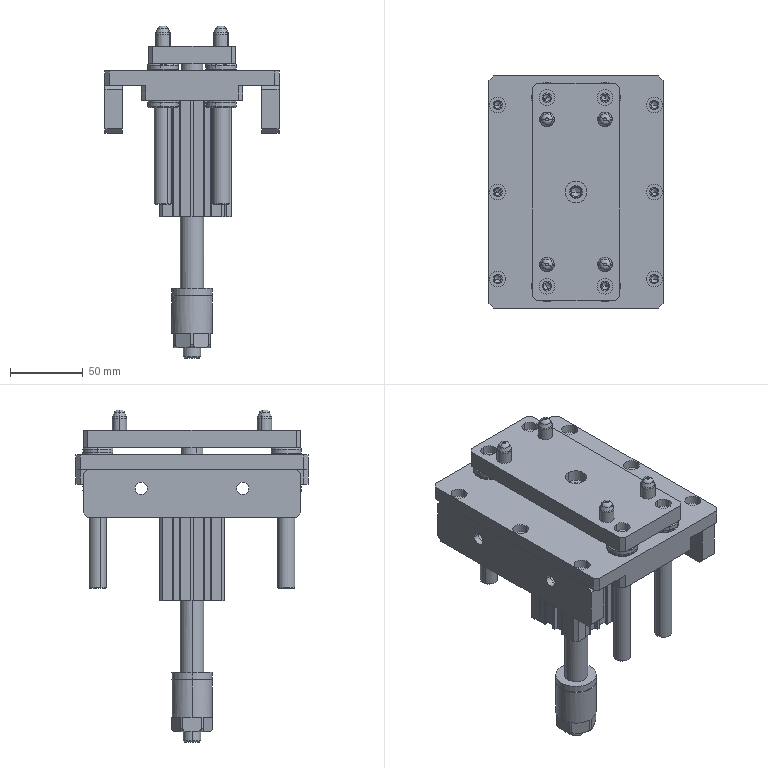Assembly | SolidWorks | mm | 20 component files | 20 solids | 847 faces | box 120 x 160 x 228.9 mm | volume 634230 mm3 | cylinder 377 | plane 268 | cone 138 | torus 48 | spline 16 | commonest cylinder face diameters 11 x36 0.4 x36 21 x32 12 x28 6.6 x24 5 x20 9 x18 10 x16
Bill of materials:
A-C13SupportCylinderBasePlate | 1 |  | Rectangular plate with chamfered corners. It has a stepped underside, a central counterbored through hole, four small holes around the center, four large counterbored holes near the ends and six small holes along the long edges.
A-C14LocatingMechanismGuidePost | 4 |  | Long slender round rod with a small axial hole at one end. It may be a hollow tube.
A-C15UpperSupportPlate | 1 |  | Long rectangular flat plate with chamfered corners. It has eight counterbored holes in two-by-two groups at each end and one central counterbored hole.
A-C17GuidePin | 4 |  | Solid cylinder with a rounded, tapered, dome-like end and a small chamfer at the opposite end.
A-C18EjectorMechanismConnectingBlock2 | 2 |  | Rectangular bar with chamfered end corners. Two larger holes pass through the wide face and three small holes are on one narrow face.
BEN | 1 |  | Square-section extruded-profile body. It has a large central bore, four corner bores, slots and grooves running along its length, a raised tab on one side, and two cross holes in one side face.
GAN | 1 |  | Stepped round shaft with a short collar section made of several flanges. It has an axial hole at one end and cross features near the ends.
TIAO | 1 |  | Cylindrical sleeve with an axial through bore and a thin circumferential line/groove near one end. The opposite end has a section with wrench-style flats.
LinearBearingLMUM12 | 4 |  | Thick-walled cylindrical bushing with an axial through bore, rounded edges, and two external circumferential grooves near the ends.
Mates:
1. coincident | A-C14LocatingMechanismGuidePost-1 face at (-53.181, -42.432, 18) dir (0, 0, 1) | A-C14LocatingMechanismGuidePost-2 face at (-53.181, 87.568, 18) dir (0, 0, 1)
2. concentric | A-C14LocatingMechanismGuidePost-1 face at (-53.181, -42.432, 18) dir (0, 0, 1) r 2.5 | A-C15UpperSupportPlate-1 face at (-53.181, -42.432, 27) dir (0, 0, 1) r 3.3
3. concentric | A-C13SupportCylinderBasePlate-1 face at (-53.181, 87.568, 10) dir (0, 0, -1) r 10.6 | LinearBearingLMUM12-1 face at (-53.181, 87.568, 14.9) dir (0, 0, -1) r 10.5
4. coincident | A-C13SupportCylinderBasePlate-1 face at (-68.181, 102.568, -10.3) dir (0, 0, -1) | LinearBearingLMUM12-1 face at (-53.181, 77.068, -10.3) dir (0, 0, -1)
5. concentric | A-C13SupportCylinderBasePlate-1 face at (-13.181, 87.568, 10) dir (0, 0, -1) r 10.6 | LinearBearingLMUM12-2 face at (-13.181, 87.568, 14.8) dir (0, 0, -1) r 10.5
6. coincident | A-C13SupportCylinderBasePlate-1 face at (-93.181, -57.432, 10) dir (0, 0, 1) | LinearBearingLMUM12-2 face at (-13.181, 77.068, 10) dir (0, 0, 1)
7. concentric | A-C13SupportCylinderBasePlate-1 face at (-13.181, -42.432, 10) dir (0, 0, -1) r 10.6 | LinearBearingLMUM12-3 face at (-13.181, -42.432, 14.8) dir (0, 0, -1) r 10.5
8. coincident | A-C13SupportCylinderBasePlate-1 face at (-93.181, -57.432, 10) dir (0, 0, 1) | LinearBearingLMUM12-3 face at (-3.281, -45.931, 10) dir (0, 0, 1)
9. concentric | A-C13SupportCylinderBasePlate-1 face at (-53.181, -42.432, 10) dir (0, 0, -1) r 10.6 | LinearBearingLMUM12-4 face at (-53.181, -42.432, 14.8) dir (0, 0, -1) r 10.5
10. coincident | A-C13SupportCylinderBasePlate-1 face at (-93.181, -57.432, 10) dir (0, 0, 1) | LinearBearingLMUM12-4 face at (-42.816, -44.114, 10) dir (0, 0, 1)
11. concentric | A-C14LocatingMechanismGuidePost-2 face at (-53.181, 87.568, -82) dir (0, 0, 1) r 6 | LinearBearingLMUM12-1 face at (-53.181, 87.568, 14.9) dir (0, 0, -1) r 6
12. concentric | A-C14LocatingMechanismGuidePost-1 face at (-53.181, -42.432, -82) dir (0, 0, 1) r 6 | LinearBearingLMUM12-4 face at (-53.181, -42.432, 14.8) dir (0, 0, -1) r 6
13. concentric | A-C14LocatingMechanismGuidePost-3 face at (-13.181, 87.568, -82) dir (0, 0, 1) r 6 | LinearBearingLMUM12-2 face at (-13.181, 87.568, 14.8) dir (0, 0, -1) r 6
14. concentric | A-C14LocatingMechanismGuidePost-4 face at (-13.181, -42.432, -82) dir (0, 0, 1) r 6 | LinearBearingLMUM12-3 face at (-13.181, -42.432, 14.8) dir (0, 0, -1) r 6
15. coincident | A-C14LocatingMechanismGuidePost-1 face at (-53.181, -42.432, 18) dir (0, 0, 1) | A-C14LocatingMechanismGuidePost-4 face at (-13.181, -42.432, 18) dir (0, 0, 1)
16. coincident | A-C14LocatingMechanismGuidePost-3 face at (-13.181, 87.568, 18) dir (0, 0, 1) | A-C14LocatingMechanismGuidePost-4 face at (-13.181, -42.432, 18) dir (0, 0, 1)
17. coincident | A-C14LocatingMechanismGuidePost-2 face at (-53.181, 87.568, 18) dir (0, 0, 1) | A-C14LocatingMechanismGuidePost-3 face at (-13.181, 87.568, 18) dir (0, 0, 1)
18. coincident | A-C14LocatingMechanismGuidePost-2 face at (-53.181, 87.568, 18) dir (0, 0, 1) | A-C15UpperSupportPlate-1 face at (-53.181, 87.568, 18) dir (0, 0, -1)
19. concentric | A-C14LocatingMechanismGuidePost-2 face at (-53.181, 87.568, -82) dir (0, 0, 1) r 6 | A-C15UpperSupportPlate-1 face at (-53.181, 87.568, 18) dir (0, 0, -1) r 6
20. concentric | A-C15UpperSupportPlate-1 face at (-53.181, 72.568, 23) dir (0, 0, 1) r 5 | A-C17GuidePin-1 face at (-53.181, 72.568, 41) dir (0, 0, -1) r 5
21. coincident | A-C15UpperSupportPlate-1 face at (-53.181, 72.568, 23) dir (0, 0, 1) | A-C17GuidePin-1 face at (-53.181, 72.568, 23) dir (0, 0, -1)
22. concentric | A-C15UpperSupportPlate-1 face at (-13.181, 72.568, 23) dir (0, 0, 1) r 5 | A-C17GuidePin-2 face at (-13.181, 72.568, 41) dir (0, 0, -1) r 5
23. coincident | A-C15UpperSupportPlate-1 face at (-13.181, 72.568, 23) dir (0, 0, 1) | A-C17GuidePin-2 face at (-13.181, 72.568, 23) dir (0, 0, -1)
24. concentric | A-C15UpperSupportPlate-1 face at (-13.181, -27.432, 23) dir (0, 0, 1) r 5 | A-C17GuidePin-4 face at (-13.181, -27.432, 41) dir (0, 0, -1) r 5
25. coincident | A-C15UpperSupportPlate-1 face at (-13.181, -27.432, 23) dir (0, 0, 1) | A-C17GuidePin-4 face at (-13.181, -27.432, 23) dir (0, 0, -1)
26. concentric | A-C15UpperSupportPlate-1 face at (-53.181, -27.432, 23) dir (0, 0, 1) r 5 | A-C17GuidePin-3 face at (-53.181, -27.432, 41) dir (0, 0, -1) r 5
27. coincident | A-C15UpperSupportPlate-1 face at (-53.181, -27.432, 23) dir (0, 0, 1) | A-C17GuidePin-3 face at (-53.181, -27.432, 23) dir (0, 0, -1)
28. coincident | A-C13SupportCylinderBasePlate-1 face at (-93.181, -57.432, 0) dir (0, 0, -1) | A-C18EjectorMechanismConnectingBlock2-1 face at (14.819, -52.432, 0) dir (0, 0, 1)
29. coincident | A-C13SupportCylinderBasePlate-1 face at (26.819, 102.568, 10) dir (1, 0, 0) | A-C18EjectorMechanismConnectingBlock2-1 face at (26.819, 97.568, 0) dir (1, 0, 0)
30. width | A-C18EjectorMechanismConnectingBlock2-1 face at (14.819, 97.568, -33) dir (0, 1, 0) | A-C18EjectorMechanismConnectingBlock2-1 face at (14.819, -52.432, -33) dir (0, -1, 0) | A-C13SupportCylinderBasePlate-1 face at (-93.181, 102.568, 10) dir (0, 1, 0) | A-C13SupportCylinderBasePlate-1 face at (-93.181, -57.432, 10) dir (0, -1, 0)
31. coincident | A-C13SupportCylinderBasePlate-1 face at (-93.181, -57.432, 0) dir (0, 0, -1) | A-C18EjectorMechanismConnectingBlock2-2 face at (-93.181, -52.432, 0) dir (0, 0, 1)
32. coincident | A-C13SupportCylinderBasePlate-1 face at (-93.181, 102.568, 10) dir (-1, 0, 0) | A-C18EjectorMechanismConnectingBlock2-2 face at (-93.181, 97.568, 0) dir (-1, 0, 0)
33. coincident | A-C18EjectorMechanismConnectingBlock2-1 face at (14.819, 97.568, -33) dir (0, 1, 0) | A-C18EjectorMechanismConnectingBlock2-2 face at (-93.181, 97.568, -33) dir (0, 1, 0)
34. coincident | A-C13SupportCylinderBasePlate-1 face at (-93.181, -57.432, 0) dir (0, 0, -1) | JDAD32x50-20-SE2-1/BEN-1 face at (-33.181, 22.568, 0) dir (0, 0, 1)
35. concentric | A-C13SupportCylinderBasePlate-1 face at (-16.181, 39.568, 10) dir (0, 0, 1) r 3.3 | JDAD32x50-20-SE2-1/BEN-1 face at (-16.181, 39.568, -31.125) dir (0, 0, -1) r 2.6
36. concentric | A-C13SupportCylinderBasePlate-1 face at (-50.181, 5.568, 10) dir (0, 0, 1) r 3.3 | JDAD32x50-20-SE2-1/BEN-1 face at (-50.181, 5.568, -12) dir (0, 0, -1) r 2.458
37. concentric | JDAD32x50-20-SE2-1/GAN-1 face at (-33.181, 22.568, -1.138) dir (0, 0, -1) r 3.324 | CylinderWasher2-1 face at (-33.181, 22.568, 15) dir (0, 0, -1) r 4.25
38. coincident | A-C15UpperSupportPlate-1 face at (-63.181, 97.568, 15) dir (0, 0, -1) | CylinderWasher2-1 face at (-33.181, 22.568, 15) dir (0, 0, 1)
39. coincident | JDAD32x50-20-SE2-1/GAN-1 face at (-33.181, 26.443, 7) dir (0, 0, 1) | CylinderWasher2-1 face at (-33.181, 22.568, 7) dir (0, 0, -1)